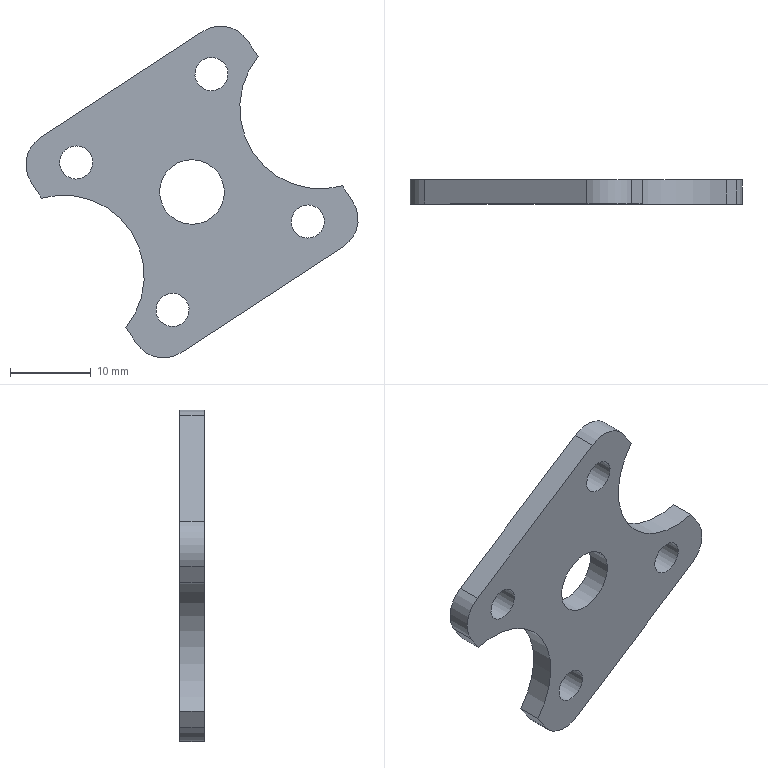Component | SolidWorks | FrontWheelSideThickPlate-2 | 1 solid | 25 faces | box 41.11 x 3 x 41.05 mm | volume 2114 mm3 | cylinder 17 | plane 8 | commonest cylinder face diameters 4.1 x8 8 x6 20 x3
build123d program:
from build123d import *

# Parameters (mm, degrees)
SKETCH1_R           = 2.05
SKETCH1_R_2         = 4
BOSS_EXTRUDE1_DEPTH = 3
FILLET1_R           = 4


with BuildPart() as part:
    # Sketch1 → Boss-Extrude1 (new body)
    with BuildSketch(Plane.XY):
        with BuildLine():
            Line((-16, -9.539), (-16, -15.9))
            Line((-16, -15.9), (16, -15.9))
            Line((16, -15.9), (16, -9.539))
            ThreePointArc((16, -9.539), (9, 0), (16, 9.539))
            Line((16, 9.539), (16, 15.9))
            Line((16, 15.9), (-16, 15.9))
            Line((-16, 15.9), (-16, 9.539))
            ThreePointArc((-16, 9.539), (-10.938, 5.916), (-9, 0))
            ThreePointArc((-9, 0), (-10.938, -5.916), (-16, -9.539))
        make_face()
        with Locations((-10, -10.9)):
            Circle(SKETCH1_R, mode=Mode.SUBTRACT)
        with Locations((10, -10.9)):
            Circle(SKETCH1_R, mode=Mode.SUBTRACT)
        with Locations((-10, 10.9)):
            Circle(SKETCH1_R, mode=Mode.SUBTRACT)
        Circle(SKETCH1_R_2, mode=Mode.SUBTRACT)
        with Locations((10, 10.9)):
            Circle(SKETCH1_R, mode=Mode.SUBTRACT)
    extrude(amount=BOSS_EXTRUDE1_DEPTH)

    # Fillet1
    fillet1_edges = [part.edges().sort_by_distance(p)[0] for p in [
        (-16, 15.9, 1.5),
        (16, 15.9, 1.5),
        (16, -15.9, 1.5),
        (-16, -15.9, 1.5),
    ]]
    fillet(fillet1_edges, radius=FILLET1_R)


solid = part.part

# Placed as in the assembly
solid = solid.moved(Location((0.3183, 23.4, 37), (-90, 0, -33.158)))
STEP:
#1=COLOUR_RGB('',0.7922,0.8196,0.9333);
#2=FILL_AREA_STYLE_COLOUR('',#1);
#3=FILL_AREA_STYLE('',(#2));
#4=SURFACE_STYLE_FILL_AREA(#3);
#5=SURFACE_SIDE_STYLE('',(#4));
#6=SURFACE_STYLE_USAGE(.BOTH.,#5);
#7=PRESENTATION_STYLE_ASSIGNMENT((#6));
#8=CARTESIAN_POINT('',(0.6444,0.9212,1.357));
#9=VERTEX_POINT('',#8);
#10=CARTESIAN_POINT('',(0.5093,0.9212,1.269));
#11=VERTEX_POINT('',#10);
#12=CARTESIAN_POINT('',(0.5768,0.9212,1.313));
#13=DIRECTION('',(0.,1.,0.));
#14=DIRECTION('',(0.8372,0.,0.5469));
#15=AXIS2_PLACEMENT_3D('',#12,#13,#14);
#16=CIRCLE('',#15,0.08071);
#17=EDGE_CURVE('',#9,#11,#16,.T.);
#18=ORIENTED_EDGE('',*,*,#17,.F.);
#19=CARTESIAN_POINT('',(0.6444,1.039,1.357));
#20=VERTEX_POINT('',#19);
#21=CARTESIAN_POINT('',(0.6444,0.9212,1.357));
#22=DIRECTION('',(0.,1.,0.));
#23=VECTOR('',#22,39.37);
#24=LINE('',#21,#23);
#25=EDGE_CURVE('',#9,#20,#24,.T.);
#26=ORIENTED_EDGE('',*,*,#25,.T.);
#27=CARTESIAN_POINT('',(0.5093,1.039,1.269));
#28=VERTEX_POINT('',#27);
#29=CARTESIAN_POINT('',(0.5768,1.039,1.313));
#30=DIRECTION('',(0.,1.,0.));
#31=DIRECTION('',(0.8372,0.,0.5469));
#32=AXIS2_PLACEMENT_3D('',#29,#30,#31);
#33=CIRCLE('',#32,0.08071);
#34=EDGE_CURVE('',#20,#28,#33,.T.);
#35=ORIENTED_EDGE('',*,*,#34,.T.);
#36=CARTESIAN_POINT('',(0.5093,0.9212,1.269));
#37=DIRECTION('',(0.,1.,0.));
#38=VECTOR('',#37,39.37);
#39=LINE('',#36,#38);
#40=EDGE_CURVE('',#11,#28,#39,.T.);
#41=ORIENTED_EDGE('',*,*,#40,.F.);
#42=EDGE_LOOP('',(#18,#26,#35,#41));
#43=FACE_OUTER_BOUND('',#42,.T.);
#44=CARTESIAN_POINT('',(0.5768,0.9212,1.313));
#45=DIRECTION('',(0.,1.,0.));
#46=DIRECTION('',(-0.8372,0.,-0.5469));
#47=AXIS2_PLACEMENT_3D('',#44,#45,#46);
#48=CYLINDRICAL_SURFACE('',#47,0.08071);
#49=ADVANCED_FACE('',(#43),#48,.F.);
#50=CARTESIAN_POINT('',(0.03985,0.9212,1.987));
#51=VERTEX_POINT('',#50);
#52=CARTESIAN_POINT('',(0.175,0.9212,2.075));
#53=VERTEX_POINT('',#52);
#54=CARTESIAN_POINT('',(0.1074,0.9212,2.031));
#55=DIRECTION('',(0.,-1.,0.));
#56=DIRECTION('',(0.8372,0.,0.5469));
#57=AXIS2_PLACEMENT_3D('',#54,#55,#56);
#58=CIRCLE('',#57,0.08071);
#59=EDGE_CURVE('',#51,#53,#58,.T.);
#60=ORIENTED_EDGE('',*,*,#59,.T.);
#61=CARTESIAN_POINT('',(0.175,1.039,2.075));
#62=VERTEX_POINT('',#61);
#63=CARTESIAN_POINT('',(0.175,0.9212,2.075));
#64=DIRECTION('',(0.,1.,0.));
#65=VECTOR('',#64,39.37);
#66=LINE('',#63,#65);
#67=EDGE_CURVE('',#53,#62,#66,.T.);
#68=ORIENTED_EDGE('',*,*,#67,.T.);
#69=CARTESIAN_POINT('',(0.03985,1.039,1.987));
#70=VERTEX_POINT('',#69);
#71=CARTESIAN_POINT('',(0.1074,1.039,2.031));
#72=DIRECTION('',(0.,-1.,0.));
#73=DIRECTION('',(0.8372,0.,0.5469));
#74=AXIS2_PLACEMENT_3D('',#71,#72,#73);
#75=CIRCLE('',#74,0.08071);
#76=EDGE_CURVE('',#70,#62,#75,.T.);
#77=ORIENTED_EDGE('',*,*,#76,.F.);
#78=CARTESIAN_POINT('',(0.03985,0.9212,1.987));
#79=DIRECTION('',(0.,1.,0.));
#80=VECTOR('',#79,39.37);
#81=LINE('',#78,#80);
#82=EDGE_CURVE('',#51,#70,#81,.T.);
#83=ORIENTED_EDGE('',*,*,#82,.F.);
#84=EDGE_LOOP('',(#60,#68,#77,#83));
#85=FACE_OUTER_BOUND('',#84,.T.);
#86=CARTESIAN_POINT('',(0.1074,0.9212,2.031));
#87=DIRECTION('',(0.,1.,0.));
#88=DIRECTION('',(-0.8372,0.,-0.5469));
#89=AXIS2_PLACEMENT_3D('',#86,#87,#88);
#90=CYLINDRICAL_SURFACE('',#89,0.08071);
#91=ADVANCED_FACE('',(#85),#90,.F.);
#92=CARTESIAN_POINT('',(-0.6193,0.9212,1.556));
#93=VERTEX_POINT('',#92);
#94=CARTESIAN_POINT('',(-0.4842,0.9212,1.645));
#95=VERTEX_POINT('',#94);
#96=CARTESIAN_POINT('',(-0.5518,0.9212,1.601));
#97=DIRECTION('',(0.,-1.,0.));
#98=DIRECTION('',(0.8372,0.,0.5469));
#99=AXIS2_PLACEMENT_3D('',#96,#97,#98);
#100=CIRCLE('',#99,0.08071);
#101=EDGE_CURVE('',#93,#95,#100,.T.);
#102=ORIENTED_EDGE('',*,*,#101,.T.);
#103=CARTESIAN_POINT('',(-0.4842,1.039,1.645));
#104=VERTEX_POINT('',#103);
#105=CARTESIAN_POINT('',(-0.4842,0.9212,1.645));
#106=DIRECTION('',(0.,1.,0.));
#107=VECTOR('',#106,39.37);
#108=LINE('',#105,#107);
#109=EDGE_CURVE('',#95,#104,#108,.T.);
#110=ORIENTED_EDGE('',*,*,#109,.T.);
#111=CARTESIAN_POINT('',(-0.6193,1.039,1.556));
#112=VERTEX_POINT('',#111);
#113=CARTESIAN_POINT('',(-0.5518,1.039,1.601));
#114=DIRECTION('',(0.,-1.,0.));
#115=DIRECTION('',(0.8372,0.,0.5469));
#116=AXIS2_PLACEMENT_3D('',#113,#114,#115);
#117=CIRCLE('',#116,0.08071);
#118=EDGE_CURVE('',#112,#104,#117,.T.);
#119=ORIENTED_EDGE('',*,*,#118,.F.);
#120=CARTESIAN_POINT('',(-0.6193,0.9212,1.556));
#121=DIRECTION('',(0.,1.,0.));
#122=VECTOR('',#121,39.37);
#123=LINE('',#120,#122);
#124=EDGE_CURVE('',#93,#112,#123,.T.);
#125=ORIENTED_EDGE('',*,*,#124,.F.);
#126=EDGE_LOOP('',(#102,#110,#119,#125));
#127=FACE_OUTER_BOUND('',#126,.T.);
#128=CARTESIAN_POINT('',(-0.5518,0.9212,1.601));
#129=DIRECTION('',(0.,1.,0.));
#130=DIRECTION('',(-0.8372,0.,-0.5469));
#131=AXIS2_PLACEMENT_3D('',#128,#129,#130);
#132=CYLINDRICAL_SURFACE('',#131,0.08071);
#133=ADVANCED_FACE('',(#127),#132,.F.);
#134=CARTESIAN_POINT('',(-0.01478,0.9212,0.9262));
#135=VERTEX_POINT('',#134);
#136=CARTESIAN_POINT('',(-0.1499,0.9212,0.838));
#137=VERTEX_POINT('',#136);
#138=CARTESIAN_POINT('',(-0.08235,0.9212,0.8821));
#139=DIRECTION('',(0.,1.,0.));
#140=DIRECTION('',(0.8372,0.,0.5469));
#141=AXIS2_PLACEMENT_3D('',#138,#139,#140);
#142=CIRCLE('',#141,0.08071);
#143=EDGE_CURVE('',#135,#137,#142,.T.);
#144=ORIENTED_EDGE('',*,*,#143,.F.);
#145=CARTESIAN_POINT('',(-0.01478,1.039,0.9262));
#146=VERTEX_POINT('',#145);
#147=CARTESIAN_POINT('',(-0.01478,0.9212,0.9262));
#148=DIRECTION('',(0.,1.,0.));
#149=VECTOR('',#148,39.37);
#150=LINE('',#147,#149);
#151=EDGE_CURVE('',#135,#146,#150,.T.);
#152=ORIENTED_EDGE('',*,*,#151,.T.);
#153=CARTESIAN_POINT('',(-0.1499,1.039,0.838));
#154=VERTEX_POINT('',#153);
#155=CARTESIAN_POINT('',(-0.08235,1.039,0.8821));
#156=DIRECTION('',(0.,1.,0.));
#157=DIRECTION('',(0.8372,0.,0.5469));
#158=AXIS2_PLACEMENT_3D('',#155,#156,#157);
#159=CIRCLE('',#158,0.08071);
#160=EDGE_CURVE('',#146,#154,#159,.T.);
#161=ORIENTED_EDGE('',*,*,#160,.T.);
#162=CARTESIAN_POINT('',(-0.1499,0.9212,0.838));
#163=DIRECTION('',(0.,1.,0.));
#164=VECTOR('',#163,39.37);
#165=LINE('',#162,#164);
#166=EDGE_CURVE('',#137,#154,#165,.T.);
#167=ORIENTED_EDGE('',*,*,#166,.F.);
#168=EDGE_LOOP('',(#144,#152,#161,#167));
#169=FACE_OUTER_BOUND('',#168,.T.);
#170=CARTESIAN_POINT('',(-0.08235,0.9212,0.8821));
#171=DIRECTION('',(0.,1.,0.));
#172=DIRECTION('',(-0.8372,0.,-0.5469));
#173=AXIS2_PLACEMENT_3D('',#170,#171,#172);
#174=CYLINDRICAL_SURFACE('',#173,0.08071);
#175=ADVANCED_FACE('',(#169),#174,.F.);
#176=CARTESIAN_POINT('',(-0.1193,0.9212,1.371));
#177=VERTEX_POINT('',#176);
#178=CARTESIAN_POINT('',(0.1444,0.9212,1.543));
#179=VERTEX_POINT('',#178);
#180=CARTESIAN_POINT('',(0.01253,0.9212,1.457));
#181=DIRECTION('',(0.,-1.,0.));
#182=DIRECTION('',(0.8372,0.,0.5469));
#183=AXIS2_PLACEMENT_3D('',#180,#181,#182);
#184=CIRCLE('',#183,0.1575);
#185=EDGE_CURVE('',#177,#179,#184,.T.);
#186=ORIENTED_EDGE('',*,*,#185,.T.);
#187=CARTESIAN_POINT('',(0.1444,1.039,1.543));
#188=VERTEX_POINT('',#187);
#189=CARTESIAN_POINT('',(0.1444,0.9212,1.543));
#190=DIRECTION('',(0.,1.,0.));
#191=VECTOR('',#190,39.37);
#192=LINE('',#189,#191);
#193=EDGE_CURVE('',#179,#188,#192,.T.);
#194=ORIENTED_EDGE('',*,*,#193,.T.);
#195=CARTESIAN_POINT('',(-0.1193,1.039,1.371));
#196=VERTEX_POINT('',#195);
#197=CARTESIAN_POINT('',(0.01253,1.039,1.457));
#198=DIRECTION('',(0.,-1.,0.));
#199=DIRECTION('',(0.8372,0.,0.5469));
#200=AXIS2_PLACEMENT_3D('',#197,#198,#199);
#201=CIRCLE('',#200,0.1575);
#202=EDGE_CURVE('',#196,#188,#201,.T.);
#203=ORIENTED_EDGE('',*,*,#202,.F.);
#204=CARTESIAN_POINT('',(-0.1193,0.9212,1.371));
#205=DIRECTION('',(0.,1.,0.));
#206=VECTOR('',#205,39.37);
#207=LINE('',#204,#206);
#208=EDGE_CURVE('',#177,#196,#207,.T.);
#209=ORIENTED_EDGE('',*,*,#208,.F.);
#210=EDGE_LOOP('',(#186,#194,#203,#209));
#211=FACE_OUTER_BOUND('',#210,.T.);
#212=CARTESIAN_POINT('',(0.01253,0.9212,1.457));
#213=DIRECTION('',(0.,1.,0.));
#214=DIRECTION('',(-0.8372,0.,-0.5469));
#215=AXIS2_PLACEMENT_3D('',#212,#213,#214);
#216=CYLINDRICAL_SURFACE('',#215,0.1575);
#217=ADVANCED_FACE('',(#211),#216,.F.);
#218=CARTESIAN_POINT('',(0.3345,0.9212,2.116));
#219=VERTEX_POINT('',#218);
#220=CARTESIAN_POINT('',(0.3092,0.9212,1.65));
#221=VERTEX_POINT('',#220);
#222=CARTESIAN_POINT('',(0.6388,0.9212,1.866));
#223=DIRECTION('',(0.,-1.,0.));
#224=DIRECTION('',(0.8372,0.,0.5469));
#225=AXIS2_PLACEMENT_3D('',#222,#223,#224);
#226=CIRCLE('',#225,0.3937);
#227=EDGE_CURVE('',#219,#221,#226,.T.);
#228=ORIENTED_EDGE('',*,*,#227,.T.);
#229=CARTESIAN_POINT('',(0.3092,1.039,1.65));
#230=VERTEX_POINT('',#229);
#231=CARTESIAN_POINT('',(0.3092,0.9212,1.65));
#232=DIRECTION('',(0.,1.,0.));
#233=VECTOR('',#232,39.37);
#234=LINE('',#231,#233);
#235=EDGE_CURVE('',#221,#230,#234,.T.);
#236=ORIENTED_EDGE('',*,*,#235,.T.);
#237=CARTESIAN_POINT('',(0.3345,1.039,2.116));
#238=VERTEX_POINT('',#237);
#239=CARTESIAN_POINT('',(0.6388,1.039,1.866));
#240=DIRECTION('',(0.,-1.,0.));
#241=DIRECTION('',(0.8372,0.,0.5469));
#242=AXIS2_PLACEMENT_3D('',#239,#240,#241);
#243=CIRCLE('',#242,0.3937);
#244=EDGE_CURVE('',#238,#230,#243,.T.);
#245=ORIENTED_EDGE('',*,*,#244,.F.);
#246=CARTESIAN_POINT('',(0.3345,0.9212,2.116));
#247=DIRECTION('',(0.,1.,0.));
#248=VECTOR('',#247,39.37);
#249=LINE('',#246,#248);
#250=EDGE_CURVE('',#219,#238,#249,.T.);
#251=ORIENTED_EDGE('',*,*,#250,.F.);
#252=EDGE_LOOP('',(#228,#236,#245,#251));
#253=FACE_OUTER_BOUND('',#252,.T.);
#254=CARTESIAN_POINT('',(0.6388,0.9212,1.866));
#255=DIRECTION('',(0.,1.,0.));
#256=DIRECTION('',(-0.8372,0.,-0.5469));
#257=AXIS2_PLACEMENT_3D('',#254,#255,#256);
#258=CYLINDRICAL_SURFACE('',#257,0.3937);
#259=ADVANCED_FACE('',(#253),#258,.F.);
#260=CARTESIAN_POINT('',(-0.7202,0.9212,1.427));
#261=VERTEX_POINT('',#260);
#262=CARTESIAN_POINT('',(-0.7711,0.9212,1.504));
#263=VERTEX_POINT('',#262);
#264=CARTESIAN_POINT('',(-0.5148,0.9212,1.112));
#265=DIRECTION('',(-0.5469,0.,0.8372));
#266=VECTOR('',#265,39.37);
#267=LINE('',#264,#266);
#268=EDGE_CURVE('',#261,#263,#267,.T.);
#269=ORIENTED_EDGE('',*,*,#268,.T.);
#270=CARTESIAN_POINT('',(-0.7711,1.039,1.504));
#271=VERTEX_POINT('',#270);
#272=CARTESIAN_POINT('',(-0.7711,0.9212,1.504));
#273=DIRECTION('',(0.,1.,0.));
#274=VECTOR('',#273,39.37);
#275=LINE('',#272,#274);
#276=EDGE_CURVE('',#263,#271,#275,.T.);
#277=ORIENTED_EDGE('',*,*,#276,.T.);
#278=CARTESIAN_POINT('',(-0.7202,1.039,1.427));
#279=VERTEX_POINT('',#278);
#280=CARTESIAN_POINT('',(-0.5148,1.039,1.112));
#281=DIRECTION('',(-0.5469,0.,0.8372));
#282=VECTOR('',#281,39.37);
#283=LINE('',#280,#282);
#284=EDGE_CURVE('',#279,#271,#283,.T.);
#285=ORIENTED_EDGE('',*,*,#284,.F.);
#286=CARTESIAN_POINT('',(-0.7202,0.9212,1.427));
#287=DIRECTION('',(0.,1.,0.));
#288=VECTOR('',#287,39.37);
#289=LINE('',#286,#288);
#290=EDGE_CURVE('',#261,#279,#289,.T.);
#291=ORIENTED_EDGE('',*,*,#290,.F.);
#292=EDGE_LOOP('',(#269,#277,#285,#291));
#293=FACE_OUTER_BOUND('',#292,.T.);
#294=CARTESIAN_POINT('',(-0.5148,0.9212,1.112));
#295=DIRECTION('',(-0.8372,0.,-0.5469));
#296=DIRECTION('',(0.,-1.,0.));
#297=AXIS2_PLACEMENT_3D('',#294,#295,#296);
#298=PLANE('',#297);
#299=ADVANCED_FACE('',(#293),#298,.T.);
#300=CARTESIAN_POINT('',(-0.3094,1.039,0.7977));
#301=VERTEX_POINT('',#300);
#302=CARTESIAN_POINT('',(-0.6137,1.039,1.048));
#303=DIRECTION('',(0.,1.,0.));
#304=DIRECTION('',(0.8372,0.,0.5469));
#305=AXIS2_PLACEMENT_3D('',#302,#303,#304);
#306=CIRCLE('',#305,0.3937);
#307=EDGE_CURVE('',#279,#301,#306,.T.);
#308=ORIENTED_EDGE('',*,*,#307,.T.);
#309=CARTESIAN_POINT('',(-0.3094,0.9212,0.7977));
#310=VERTEX_POINT('',#309);
#311=CARTESIAN_POINT('',(-0.3094,0.9212,0.7977));
#312=DIRECTION('',(0.,1.,0.));
#313=VECTOR('',#312,39.37);
#314=LINE('',#311,#313);
#315=EDGE_CURVE('',#310,#301,#314,.T.);
#316=ORIENTED_EDGE('',*,*,#315,.F.);
#317=CARTESIAN_POINT('',(-0.6137,0.9212,1.048));
#318=DIRECTION('',(0.,1.,0.));
#319=DIRECTION('',(0.8372,0.,0.5469));
#320=AXIS2_PLACEMENT_3D('',#317,#318,#319);
#321=CIRCLE('',#320,0.3937);
#322=EDGE_CURVE('',#261,#310,#321,.T.);
#323=ORIENTED_EDGE('',*,*,#322,.F.);
#324=ORIENTED_EDGE('',*,*,#290,.T.);
#325=EDGE_LOOP('',(#308,#316,#323,#324));
#326=FACE_OUTER_BOUND('',#325,.T.);
#327=CARTESIAN_POINT('',(-0.6137,0.9212,1.048));
#328=DIRECTION('',(0.,1.,0.));
#329=DIRECTION('',(-0.8372,0.,-0.5469));
#330=AXIS2_PLACEMENT_3D('',#327,#328,#329);
#331=CYLINDRICAL_SURFACE('',#330,0.3937);
#332=ADVANCED_FACE('',(#326),#331,.F.);
#333=CARTESIAN_POINT('',(-0.2586,1.039,0.7199));
#334=VERTEX_POINT('',#333);
#335=CARTESIAN_POINT('',(-0.5148,1.039,1.112));
#336=DIRECTION('',(-0.5469,0.,0.8372));
#337=VECTOR('',#336,39.37);
#338=LINE('',#335,#337);
#339=EDGE_CURVE('',#334,#301,#338,.T.);
#340=ORIENTED_EDGE('',*,*,#339,.F.);
#341=CARTESIAN_POINT('',(-0.2586,0.9212,0.7199));
#342=VERTEX_POINT('',#341);
#343=CARTESIAN_POINT('',(-0.2586,0.9212,0.7199));
#344=DIRECTION('',(0.,-1.,0.));
#345=VECTOR('',#344,39.37);
#346=LINE('',#343,#345);
#347=EDGE_CURVE('',#334,#342,#346,.T.);
#348=ORIENTED_EDGE('',*,*,#347,.T.);
#349=CARTESIAN_POINT('',(-0.5148,0.9212,1.112));
#350=DIRECTION('',(-0.5469,0.,0.8372));
#351=VECTOR('',#350,39.37);
#352=LINE('',#349,#351);
#353=EDGE_CURVE('',#342,#310,#352,.T.);
#354=ORIENTED_EDGE('',*,*,#353,.T.);
#355=ORIENTED_EDGE('',*,*,#315,.T.);
#356=EDGE_LOOP('',(#340,#348,#354,#355));
#357=FACE_OUTER_BOUND('',#356,.T.);
#358=CARTESIAN_POINT('',(-0.5148,0.9212,1.112));
#359=DIRECTION('',(-0.8372,0.,-0.5469));
#360=DIRECTION('',(0.,-1.,0.));
#361=AXIS2_PLACEMENT_3D('',#358,#359,#360);
#362=PLANE('',#361);
#363=ADVANCED_FACE('',(#357),#362,.T.);
#364=CARTESIAN_POINT('',(-0.0406,0.9212,0.6742));
#365=VERTEX_POINT('',#364);
#366=CARTESIAN_POINT('',(0.7504,0.9212,1.191));
#367=VERTEX_POINT('',#366);
#368=CARTESIAN_POINT('',(0.3549,0.9212,0.9326));
#369=DIRECTION('',(0.8372,0.,0.5469));
#370=VECTOR('',#369,39.37);
#371=LINE('',#368,#370);
#372=EDGE_CURVE('',#365,#367,#371,.T.);
#373=ORIENTED_EDGE('',*,*,#372,.F.);
#374=CARTESIAN_POINT('',(-0.0406,1.039,0.6742));
#375=VERTEX_POINT('',#374);
#376=CARTESIAN_POINT('',(-0.0406,1.039,0.6742));
#377=DIRECTION('',(0.,1.,0.));
#378=VECTOR('',#377,39.37);
#379=LINE('',#376,#378);
#380=EDGE_CURVE('',#365,#375,#379,.T.);
#381=ORIENTED_EDGE('',*,*,#380,.T.);
#382=CARTESIAN_POINT('',(0.7504,1.039,1.191));
#383=VERTEX_POINT('',#382);
#384=CARTESIAN_POINT('',(0.3549,1.039,0.9326));
#385=DIRECTION('',(0.8372,0.,0.5469));
#386=VECTOR('',#385,39.37);
#387=LINE('',#384,#386);
#388=EDGE_CURVE('',#375,#383,#387,.T.);
#389=ORIENTED_EDGE('',*,*,#388,.T.);
#390=CARTESIAN_POINT('',(0.7504,0.9212,1.191));
#391=DIRECTION('',(0.,-1.,0.));
#392=VECTOR('',#391,39.37);
#393=LINE('',#390,#392);
#394=EDGE_CURVE('',#383,#367,#393,.T.);
#395=ORIENTED_EDGE('',*,*,#394,.T.);
#396=EDGE_LOOP('',(#373,#381,#389,#395));
#397=FACE_OUTER_BOUND('',#396,.T.);
#398=CARTESIAN_POINT('',(0.3549,0.9212,0.9326));
#399=DIRECTION('',(-0.5469,0.,0.8372));
#400=DIRECTION('',(-0.8372,0.,-0.5469));
#401=AXIS2_PLACEMENT_3D('',#398,#399,#400);
#402=PLANE('',#401);
#403=ADVANCED_FACE('',(#397),#402,.F.);
#404=CARTESIAN_POINT('',(0.7961,0.9212,1.409));
#405=VERTEX_POINT('',#404);
#406=CARTESIAN_POINT('',(0.7453,0.9212,1.487));
#407=VERTEX_POINT('',#406);
#408=CARTESIAN_POINT('',(0.5399,0.9212,1.801));
#409=DIRECTION('',(-0.5469,0.,0.8372));
#410=VECTOR('',#409,39.37);
#411=LINE('',#408,#410);
#412=EDGE_CURVE('',#405,#407,#411,.T.);
#413=ORIENTED_EDGE('',*,*,#412,.F.);
#414=CARTESIAN_POINT('',(0.7961,1.039,1.409));
#415=VERTEX_POINT('',#414);
#416=CARTESIAN_POINT('',(0.7961,0.9212,1.409));
#417=DIRECTION('',(0.,1.,0.));
#418=VECTOR('',#417,39.37);
#419=LINE('',#416,#418);
#420=EDGE_CURVE('',#405,#415,#419,.T.);
#421=ORIENTED_EDGE('',*,*,#420,.T.);
#422=CARTESIAN_POINT('',(0.7453,1.039,1.487));
#423=VERTEX_POINT('',#422);
#424=CARTESIAN_POINT('',(0.5399,1.039,1.801));
#425=DIRECTION('',(-0.5469,0.,0.8372));
#426=VECTOR('',#425,39.37);
#427=LINE('',#424,#426);
#428=EDGE_CURVE('',#415,#423,#427,.T.);
#429=ORIENTED_EDGE('',*,*,#428,.T.);
#430=CARTESIAN_POINT('',(0.7453,0.9212,1.487));
#431=DIRECTION('',(0.,1.,0.));
#432=VECTOR('',#431,39.37);
#433=LINE('',#430,#432);
#434=EDGE_CURVE('',#407,#423,#433,.T.);
#435=ORIENTED_EDGE('',*,*,#434,.F.);
#436=EDGE_LOOP('',(#413,#421,#429,#435));
#437=FACE_OUTER_BOUND('',#436,.T.);
#438=CARTESIAN_POINT('',(0.5399,0.9212,1.801));
#439=DIRECTION('',(-0.8372,0.,-0.5469));
#440=DIRECTION('',(0.5469,0.,-0.8372));
#441=AXIS2_PLACEMENT_3D('',#438,#439,#440);
#442=PLANE('',#441);
#443=ADVANCED_FACE('',(#437),#442,.F.);
#444=ORIENTED_EDGE('',*,*,#235,.F.);
#445=CARTESIAN_POINT('',(0.6388,0.9212,1.866));
#446=DIRECTION('',(0.,-1.,0.));
#447=DIRECTION('',(0.8372,0.,0.5469));
#448=AXIS2_PLACEMENT_3D('',#445,#446,#447);
#449=CIRCLE('',#448,0.3937);
#450=EDGE_CURVE('',#221,#407,#449,.T.);
#451=ORIENTED_EDGE('',*,*,#450,.T.);
#452=ORIENTED_EDGE('',*,*,#434,.T.);
#453=CARTESIAN_POINT('',(0.6388,1.039,1.866));
#454=DIRECTION('',(0.,-1.,0.));
#455=DIRECTION('',(0.8372,0.,0.5469));
#456=AXIS2_PLACEMENT_3D('',#453,#454,#455);
#457=CIRCLE('',#456,0.3937);
#458=EDGE_CURVE('',#230,#423,#457,.T.);
#459=ORIENTED_EDGE('',*,*,#458,.F.);
#460=EDGE_LOOP('',(#444,#451,#452,#459));
#461=FACE_OUTER_BOUND('',#460,.T.);
#462=CARTESIAN_POINT('',(0.6388,0.9212,1.866));
#463=DIRECTION('',(0.,1.,0.));
#464=DIRECTION('',(-0.8372,0.,-0.5469));
#465=AXIS2_PLACEMENT_3D('',#462,#463,#464);
#466=CYLINDRICAL_SURFACE('',#465,0.3937);
#467=ADVANCED_FACE('',(#461),#466,.F.);
#468=CARTESIAN_POINT('',(0.2836,1.039,2.193));
#469=VERTEX_POINT('',#468);
#470=CARTESIAN_POINT('',(0.5399,1.039,1.801));
#471=DIRECTION('',(-0.5469,0.,0.8372));
#472=VECTOR('',#471,39.37);
#473=LINE('',#470,#472);
#474=EDGE_CURVE('',#238,#469,#473,.T.);
#475=ORIENTED_EDGE('',*,*,#474,.T.);
#476=CARTESIAN_POINT('',(0.2836,0.9212,2.193));
#477=VERTEX_POINT('',#476);
#478=CARTESIAN_POINT('',(0.2836,0.9212,2.193));
#479=DIRECTION('',(0.,-1.,0.));
#480=VECTOR('',#479,39.37);
#481=LINE('',#478,#480);
#482=EDGE_CURVE('',#469,#477,#481,.T.);
#483=ORIENTED_EDGE('',*,*,#482,.T.);
#484=CARTESIAN_POINT('',(0.5399,0.9212,1.801));
#485=DIRECTION('',(-0.5469,0.,0.8372));
#486=VECTOR('',#485,39.37);
#487=LINE('',#484,#486);
#488=EDGE_CURVE('',#219,#477,#487,.T.);
#489=ORIENTED_EDGE('',*,*,#488,.F.);
#490=ORIENTED_EDGE('',*,*,#250,.T.);
#491=EDGE_LOOP('',(#475,#483,#489,#490));
#492=FACE_OUTER_BOUND('',#491,.T.);
#493=CARTESIAN_POINT('',(0.5399,0.9212,1.801));
#494=DIRECTION('',(-0.8372,0.,-0.5469));
#495=DIRECTION('',(0.5469,0.,-0.8372));
#496=AXIS2_PLACEMENT_3D('',#493,#494,#495);
#497=PLANE('',#496);
#498=ADVANCED_FACE('',(#492),#497,.F.);
#499=ORIENTED_EDGE('',*,*,#193,.F.);
#500=CARTESIAN_POINT('',(0.01253,0.9212,1.457));
#501=DIRECTION('',(0.,-1.,0.));
#502=DIRECTION('',(0.8372,0.,0.5469));
#503=AXIS2_PLACEMENT_3D('',#500,#501,#502);
#504=CIRCLE('',#503,0.1575);
#505=EDGE_CURVE('',#179,#177,#504,.T.);
#506=ORIENTED_EDGE('',*,*,#505,.T.);
#507=ORIENTED_EDGE('',*,*,#208,.T.);
#508=CARTESIAN_POINT('',(0.01253,1.039,1.457));
#509=DIRECTION('',(0.,-1.,0.));
#510=DIRECTION('',(0.8372,0.,0.5469));
#511=AXIS2_PLACEMENT_3D('',#508,#509,#510);
#512=CIRCLE('',#511,0.1575);
#513=EDGE_CURVE('',#188,#196,#512,.T.);
#514=ORIENTED_EDGE('',*,*,#513,.F.);
#515=EDGE_LOOP('',(#499,#506,#507,#514));
#516=FACE_OUTER_BOUND('',#515,.T.);
#517=CARTESIAN_POINT('',(0.01253,0.9212,1.457));
#518=DIRECTION('',(0.,1.,0.));
#519=DIRECTION('',(-0.8372,0.,-0.5469));
#520=AXIS2_PLACEMENT_3D('',#517,#518,#519);
#521=CYLINDRICAL_SURFACE('',#520,0.1575);
#522=ADVANCED_FACE('',(#516),#521,.F.);
#523=ORIENTED_EDGE('',*,*,#151,.F.);
#524=CARTESIAN_POINT('',(-0.08235,0.9212,0.8821));
#525=DIRECTION('',(0.,1.,0.));
#526=DIRECTION('',(0.8372,0.,0.5469));
#527=AXIS2_PLACEMENT_3D('',#524,#525,#526);
#528=CIRCLE('',#527,0.08071);
#529=EDGE_CURVE('',#137,#135,#528,.T.);
#530=ORIENTED_EDGE('',*,*,#529,.F.);
#531=ORIENTED_EDGE('',*,*,#166,.T.);
#532=CARTESIAN_POINT('',(-0.08235,1.039,0.8821));
#533=DIRECTION('',(0.,1.,0.));
#534=DIRECTION('',(0.8372,0.,0.5469));
#535=AXIS2_PLACEMENT_3D('',#532,#533,#534);
#536=CIRCLE('',#535,0.08071);
#537=EDGE_CURVE('',#154,#146,#536,.T.);
#538=ORIENTED_EDGE('',*,*,#537,.T.);
#539=EDGE_LOOP('',(#523,#530,#531,#538));
#540=FACE_OUTER_BOUND('',#539,.T.);
#541=CARTESIAN_POINT('',(-0.08235,0.9212,0.8821));
#542=DIRECTION('',(0.,1.,0.));
#543=DIRECTION('',(-0.8372,0.,-0.5469));
#544=AXIS2_PLACEMENT_3D('',#541,#542,#543);
#545=CYLINDRICAL_SURFACE('',#544,0.08071);
#546=ADVANCED_FACE('',(#540),#545,.F.);
#547=ORIENTED_EDGE('',*,*,#109,.F.);
#548=CARTESIAN_POINT('',(-0.5518,0.9212,1.601));
#549=DIRECTION('',(0.,-1.,0.));
#550=DIRECTION('',(0.8372,0.,0.5469));
#551=AXIS2_PLACEMENT_3D('',#548,#549,#550);
#552=CIRCLE('',#551,0.08071);
#553=EDGE_CURVE('',#95,#93,#552,.T.);
#554=ORIENTED_EDGE('',*,*,#553,.T.);
#555=ORIENTED_EDGE('',*,*,#124,.T.);
#556=CARTESIAN_POINT('',(-0.5518,1.039,1.601));
#557=DIRECTION('',(0.,-1.,0.));
#558=DIRECTION('',(0.8372,0.,0.5469));
#559=AXIS2_PLACEMENT_3D('',#556,#557,#558);
#560=CIRCLE('',#559,0.08071);
#561=EDGE_CURVE('',#104,#112,#560,.T.);
#562=ORIENTED_EDGE('',*,*,#561,.F.);
#563=EDGE_LOOP('',(#547,#554,#555,#562));
#564=FACE_OUTER_BOUND('',#563,.T.);
#565=CARTESIAN_POINT('',(-0.5518,0.9212,1.601));
#566=DIRECTION('',(0.,1.,0.));
#567=DIRECTION('',(-0.8372,0.,-0.5469));
#568=AXIS2_PLACEMENT_3D('',#565,#566,#567);
#569=CYLINDRICAL_SURFACE('',#568,0.08071);
#570=ADVANCED_FACE('',(#564),#569,.F.);
#571=ORIENTED_EDGE('',*,*,#67,.F.);
#572=CARTESIAN_POINT('',(0.1074,0.9212,2.031));
#573=DIRECTION('',(0.,-1.,0.));
#574=DIRECTION('',(0.8372,0.,0.5469));
#575=AXIS2_PLACEMENT_3D('',#572,#573,#574);
#576=CIRCLE('',#575,0.08071);
#577=EDGE_CURVE('',#53,#51,#576,.T.);
#578=ORIENTED_EDGE('',*,*,#577,.T.);
#579=ORIENTED_EDGE('',*,*,#82,.T.);
#580=CARTESIAN_POINT('',(0.1074,1.039,2.031));
#581=DIRECTION('',(0.,-1.,0.));
#582=DIRECTION('',(0.8372,0.,0.5469));
#583=AXIS2_PLACEMENT_3D('',#580,#581,#582);
#584=CIRCLE('',#583,0.08071);
#585=EDGE_CURVE('',#62,#70,#584,.T.);
#586=ORIENTED_EDGE('',*,*,#585,.F.);
#587=EDGE_LOOP('',(#571,#578,#579,#586));
#588=FACE_OUTER_BOUND('',#587,.T.);
#589=CARTESIAN_POINT('',(0.1074,0.9212,2.031));
#590=DIRECTION('',(0.,1.,0.));
#591=DIRECTION('',(-0.8372,0.,-0.5469));
#592=AXIS2_PLACEMENT_3D('',#589,#590,#591);
#593=CYLINDRICAL_SURFACE('',#592,0.08071);
#594=ADVANCED_FACE('',(#588),#593,.F.);
#595=ORIENTED_EDGE('',*,*,#25,.F.);
#596=CARTESIAN_POINT('',(0.5768,0.9212,1.313));
#597=DIRECTION('',(0.,1.,0.));
#598=DIRECTION('',(0.8372,0.,0.5469));
#599=AXIS2_PLACEMENT_3D('',#596,#597,#598);
#600=CIRCLE('',#599,0.08071);
#601=EDGE_CURVE('',#11,#9,#600,.T.);
#602=ORIENTED_EDGE('',*,*,#601,.F.);
#603=ORIENTED_EDGE('',*,*,#40,.T.);
#604=CARTESIAN_POINT('',(0.5768,1.039,1.313));
#605=DIRECTION('',(0.,1.,0.));
#606=DIRECTION('',(0.8372,0.,0.5469));
#607=AXIS2_PLACEMENT_3D('',#604,#605,#606);
#608=CIRCLE('',#607,0.08071);
#609=EDGE_CURVE('',#28,#20,#608,.T.);
#610=ORIENTED_EDGE('',*,*,#609,.T.);
#611=EDGE_LOOP('',(#595,#602,#603,#610));
#612=FACE_OUTER_BOUND('',#611,.T.);
#613=CARTESIAN_POINT('',(0.5768,0.9212,1.313));
#614=DIRECTION('',(0.,1.,0.));
#615=DIRECTION('',(-0.8372,0.,-0.5469));
#616=AXIS2_PLACEMENT_3D('',#613,#614,#615);
#617=CYLINDRICAL_SURFACE('',#616,0.08071);
#618=ADVANCED_FACE('',(#612),#617,.F.);
#619=CARTESIAN_POINT('',(-0.7254,0.9212,1.722));
#620=VERTEX_POINT('',#619);
#621=CARTESIAN_POINT('',(0.06567,0.9212,2.239));
#622=VERTEX_POINT('',#621);
#623=CARTESIAN_POINT('',(-0.3298,0.9212,1.981));
#624=DIRECTION('',(0.8372,0.,0.5469));
#625=VECTOR('',#624,39.37);
#626=LINE('',#623,#625);
#627=EDGE_CURVE('',#620,#622,#626,.T.);
#628=ORIENTED_EDGE('',*,*,#627,.T.);
#629=CARTESIAN_POINT('',(0.06567,1.039,2.239));
#630=VERTEX_POINT('',#629);
#631=CARTESIAN_POINT('',(0.06567,1.039,2.239));
#632=DIRECTION('',(0.,1.,0.));
#633=VECTOR('',#632,39.37);
#634=LINE('',#631,#633);
#635=EDGE_CURVE('',#622,#630,#634,.T.);
#636=ORIENTED_EDGE('',*,*,#635,.T.);
#637=CARTESIAN_POINT('',(-0.7254,1.039,1.722));
#638=VERTEX_POINT('',#637);
#639=CARTESIAN_POINT('',(-0.3298,1.039,1.981));
#640=DIRECTION('',(0.8372,0.,0.5469));
#641=VECTOR('',#640,39.37);
#642=LINE('',#639,#641);
#643=EDGE_CURVE('',#638,#630,#642,.T.);
#644=ORIENTED_EDGE('',*,*,#643,.F.);
#645=CARTESIAN_POINT('',(-0.7254,0.9212,1.722));
#646=DIRECTION('',(0.,-1.,0.));
#647=VECTOR('',#646,39.37);
#648=LINE('',#645,#647);
#649=EDGE_CURVE('',#638,#620,#648,.T.);
#650=ORIENTED_EDGE('',*,*,#649,.T.);
#651=EDGE_LOOP('',(#628,#636,#644,#650));
#652=FACE_OUTER_BOUND('',#651,.T.);
#653=CARTESIAN_POINT('',(-0.3298,0.9212,1.981));
#654=DIRECTION('',(-0.5469,0.,0.8372));
#655=DIRECTION('',(-0.8372,0.,-0.5469));
#656=AXIS2_PLACEMENT_3D('',#653,#654,#655);
#657=PLANE('',#656);
#658=ADVANCED_FACE('',(#652),#657,.T.);
#659=ORIENTED_EDGE('',*,*,#601,.T.);
#660=ORIENTED_EDGE('',*,*,#17,.T.);
#661=EDGE_LOOP('',(#659,#660));
#662=FACE_BOUND('',#661,.T.);
#663=ORIENTED_EDGE('',*,*,#59,.F.);
#664=ORIENTED_EDGE('',*,*,#577,.F.);
#665=EDGE_LOOP('',(#663,#664));
#666=FACE_BOUND('',#665,.T.);
#667=ORIENTED_EDGE('',*,*,#101,.F.);
#668=ORIENTED_EDGE('',*,*,#553,.F.);
#669=EDGE_LOOP('',(#667,#668));
#670=FACE_BOUND('',#669,.T.);
#671=ORIENTED_EDGE('',*,*,#529,.T.);
#672=ORIENTED_EDGE('',*,*,#143,.T.);
#673=EDGE_LOOP('',(#671,#672));
#674=FACE_BOUND('',#673,.T.);
#675=ORIENTED_EDGE('',*,*,#185,.F.);
#676=ORIENTED_EDGE('',*,*,#505,.F.);
#677=EDGE_LOOP('',(#675,#676));
#678=FACE_BOUND('',#677,.T.);
#679=ORIENTED_EDGE('',*,*,#353,.F.);
#680=CARTESIAN_POINT('',(-0.1267,0.9212,0.8061));
#681=DIRECTION('',(0.,-1.,0.));
#682=DIRECTION('',(0.8372,0.,0.5469));
#683=AXIS2_PLACEMENT_3D('',#680,#681,#682);
#684=CIRCLE('',#683,0.1575);
#685=EDGE_CURVE('',#342,#365,#684,.T.);
#686=ORIENTED_EDGE('',*,*,#685,.T.);
#687=ORIENTED_EDGE('',*,*,#372,.T.);
#688=CARTESIAN_POINT('',(0.6643,0.9212,1.323));
#689=DIRECTION('',(0.,-1.,0.));
#690=DIRECTION('',(0.8372,0.,0.5469));
#691=AXIS2_PLACEMENT_3D('',#688,#689,#690);
#692=CIRCLE('',#691,0.1575);
#693=EDGE_CURVE('',#367,#405,#692,.T.);
#694=ORIENTED_EDGE('',*,*,#693,.T.);
#695=ORIENTED_EDGE('',*,*,#412,.T.);
#696=ORIENTED_EDGE('',*,*,#450,.F.);
#697=ORIENTED_EDGE('',*,*,#227,.F.);
#698=ORIENTED_EDGE('',*,*,#488,.T.);
#699=CARTESIAN_POINT('',(0.1518,0.9212,2.107));
#700=DIRECTION('',(0.,-1.,0.));
#701=DIRECTION('',(0.8372,0.,0.5469));
#702=AXIS2_PLACEMENT_3D('',#699,#700,#701);
#703=CIRCLE('',#702,0.1575);
#704=EDGE_CURVE('',#477,#622,#703,.T.);
#705=ORIENTED_EDGE('',*,*,#704,.T.);
#706=ORIENTED_EDGE('',*,*,#627,.F.);
#707=CARTESIAN_POINT('',(-0.6392,0.9212,1.591));
#708=DIRECTION('',(0.,-1.,0.));
#709=DIRECTION('',(0.8372,0.,0.5469));
#710=AXIS2_PLACEMENT_3D('',#707,#708,#709);
#711=CIRCLE('',#710,0.1575);
#712=EDGE_CURVE('',#620,#263,#711,.T.);
#713=ORIENTED_EDGE('',*,*,#712,.T.);
#714=ORIENTED_EDGE('',*,*,#268,.F.);
#715=ORIENTED_EDGE('',*,*,#322,.T.);
#716=EDGE_LOOP('',(#679,#686,#687,#694,#695,#696,#697,#698,#705,#706,#713,#714,#715));
#717=FACE_OUTER_BOUND('',#716,.T.);
#718=CARTESIAN_POINT('',(0.01253,0.9212,1.457));
#719=DIRECTION('',(0.,-1.,0.));
#720=DIRECTION('',(0.8372,0.,0.5469));
#721=AXIS2_PLACEMENT_3D('',#718,#719,#720);
#722=PLANE('',#721);
#723=ADVANCED_FACE('',(#662,#666,#670,#674,#678,#717),#722,.T.);
#724=ORIENTED_EDGE('',*,*,#609,.F.);
#725=ORIENTED_EDGE('',*,*,#34,.F.);
#726=EDGE_LOOP('',(#724,#725));
#727=FACE_BOUND('',#726,.T.);
#728=ORIENTED_EDGE('',*,*,#76,.T.);
#729=ORIENTED_EDGE('',*,*,#585,.T.);
#730=EDGE_LOOP('',(#728,#729));
#731=FACE_BOUND('',#730,.T.);
#732=ORIENTED_EDGE('',*,*,#118,.T.);
#733=ORIENTED_EDGE('',*,*,#561,.T.);
#734=EDGE_LOOP('',(#732,#733));
#735=FACE_BOUND('',#734,.T.);
#736=ORIENTED_EDGE('',*,*,#537,.F.);
#737=ORIENTED_EDGE('',*,*,#160,.F.);
#738=EDGE_LOOP('',(#736,#737));
#739=FACE_BOUND('',#738,.T.);
#740=ORIENTED_EDGE('',*,*,#202,.T.);
#741=ORIENTED_EDGE('',*,*,#513,.T.);
#742=EDGE_LOOP('',(#740,#741));
#743=FACE_BOUND('',#742,.T.);
#744=ORIENTED_EDGE('',*,*,#388,.F.);
#745=CARTESIAN_POINT('',(-0.1267,1.039,0.8061));
#746=DIRECTION('',(0.,1.,0.));
#747=DIRECTION('',(0.8372,0.,0.5469));
#748=AXIS2_PLACEMENT_3D('',#745,#746,#747);
#749=CIRCLE('',#748,0.1575);
#750=EDGE_CURVE('',#375,#334,#749,.T.);
#751=ORIENTED_EDGE('',*,*,#750,.T.);
#752=ORIENTED_EDGE('',*,*,#339,.T.);
#753=ORIENTED_EDGE('',*,*,#307,.F.);
#754=ORIENTED_EDGE('',*,*,#284,.T.);
#755=CARTESIAN_POINT('',(-0.6392,1.039,1.591));
#756=DIRECTION('',(0.,1.,0.));
#757=DIRECTION('',(0.8372,0.,0.5469));
#758=AXIS2_PLACEMENT_3D('',#755,#756,#757);
#759=CIRCLE('',#758,0.1575);
#760=EDGE_CURVE('',#271,#638,#759,.T.);
#761=ORIENTED_EDGE('',*,*,#760,.T.);
#762=ORIENTED_EDGE('',*,*,#643,.T.);
#763=CARTESIAN_POINT('',(0.1518,1.039,2.107));
#764=DIRECTION('',(0.,1.,0.));
#765=DIRECTION('',(0.8372,0.,0.5469));
#766=AXIS2_PLACEMENT_3D('',#763,#764,#765);
#767=CIRCLE('',#766,0.1575);
#768=EDGE_CURVE('',#630,#469,#767,.T.);
#769=ORIENTED_EDGE('',*,*,#768,.T.);
#770=ORIENTED_EDGE('',*,*,#474,.F.);
#771=ORIENTED_EDGE('',*,*,#244,.T.);
#772=ORIENTED_EDGE('',*,*,#458,.T.);
#773=ORIENTED_EDGE('',*,*,#428,.F.);
#774=CARTESIAN_POINT('',(0.6643,1.039,1.323));
#775=DIRECTION('',(0.,1.,0.));
#776=DIRECTION('',(0.8372,0.,0.5469));
#777=AXIS2_PLACEMENT_3D('',#774,#775,#776);
#778=CIRCLE('',#777,0.1575);
#779=EDGE_CURVE('',#415,#383,#778,.T.);
#780=ORIENTED_EDGE('',*,*,#779,.T.);
#781=EDGE_LOOP('',(#744,#751,#752,#753,#754,#761,#762,#769,#770,#771,#772,#773,#780));
#782=FACE_OUTER_BOUND('',#781,.T.);
#783=CARTESIAN_POINT('',(0.01253,1.039,1.457));
#784=DIRECTION('',(0.,-1.,0.));
#785=DIRECTION('',(0.8372,0.,0.5469));
#786=AXIS2_PLACEMENT_3D('',#783,#784,#785);
#787=PLANE('',#786);
#788=ADVANCED_FACE('',(#727,#731,#735,#739,#743,#782),#787,.F.);
#789=ORIENTED_EDGE('',*,*,#685,.F.);
#790=ORIENTED_EDGE('',*,*,#347,.F.);
#791=ORIENTED_EDGE('',*,*,#750,.F.);
#792=ORIENTED_EDGE('',*,*,#380,.F.);
#793=EDGE_LOOP('',(#789,#790,#791,#792));
#794=FACE_OUTER_BOUND('',#793,.T.);
#795=CARTESIAN_POINT('',(-0.1267,0.9212,0.8061));
#796=DIRECTION('',(0.,-1.,0.));
#797=DIRECTION('',(0.8372,0.,0.5469));
#798=AXIS2_PLACEMENT_3D('',#795,#796,#797);
#799=CYLINDRICAL_SURFACE('',#798,0.1575);
#800=ADVANCED_FACE('',(#794),#799,.T.);
#801=ORIENTED_EDGE('',*,*,#693,.F.);
#802=ORIENTED_EDGE('',*,*,#394,.F.);
#803=ORIENTED_EDGE('',*,*,#779,.F.);
#804=ORIENTED_EDGE('',*,*,#420,.F.);
#805=EDGE_LOOP('',(#801,#802,#803,#804));
#806=FACE_OUTER_BOUND('',#805,.T.);
#807=CARTESIAN_POINT('',(0.6643,0.9212,1.323));
#808=DIRECTION('',(0.,1.,0.));
#809=DIRECTION('',(-0.8372,0.,-0.5469));
#810=AXIS2_PLACEMENT_3D('',#807,#808,#809);
#811=CYLINDRICAL_SURFACE('',#810,0.1575);
#812=ADVANCED_FACE('',(#806),#811,.T.);
#813=ORIENTED_EDGE('',*,*,#704,.F.);
#814=ORIENTED_EDGE('',*,*,#482,.F.);
#815=ORIENTED_EDGE('',*,*,#768,.F.);
#816=ORIENTED_EDGE('',*,*,#635,.F.);
#817=EDGE_LOOP('',(#813,#814,#815,#816));
#818=FACE_OUTER_BOUND('',#817,.T.);
#819=CARTESIAN_POINT('',(0.1518,0.9212,2.107));
#820=DIRECTION('',(0.,-1.,0.));
#821=DIRECTION('',(0.8372,0.,0.5469));
#822=AXIS2_PLACEMENT_3D('',#819,#820,#821);
#823=CYLINDRICAL_SURFACE('',#822,0.1575);
#824=ADVANCED_FACE('',(#818),#823,.T.);
#825=ORIENTED_EDGE('',*,*,#712,.F.);
#826=ORIENTED_EDGE('',*,*,#649,.F.);
#827=ORIENTED_EDGE('',*,*,#760,.F.);
#828=ORIENTED_EDGE('',*,*,#276,.F.);
#829=EDGE_LOOP('',(#825,#826,#827,#828));
#830=FACE_OUTER_BOUND('',#829,.T.);
#831=CARTESIAN_POINT('',(-0.6392,0.9212,1.591));
#832=DIRECTION('',(0.,1.,0.));
#833=DIRECTION('',(-0.8372,0.,-0.5469));
#834=AXIS2_PLACEMENT_3D('',#831,#832,#833);
#835=CYLINDRICAL_SURFACE('',#834,0.1575);
#836=ADVANCED_FACE('',(#830),#835,.T.);
#837=CLOSED_SHELL('',(#49,#91,#133,#175,#217,#259,#299,#332,#363,#403,#443,#467,#498,#522,#546,#570,#594,#618,#658,#723,#788,#800,#812,#824,#836));
#838=MANIFOLD_SOLID_BREP('',#837);
#839=STYLED_ITEM('',(#7),#838);
#840=(LENGTH_UNIT()NAMED_UNIT(*)SI_UNIT($,.METRE.));
#841=LENGTH_MEASURE_WITH_UNIT(LENGTH_MEASURE(0.0254),#840);
#842=DIMENSIONAL_EXPONENTS(1.,0.,0.,0.,0.,0.,0.);
#843=(CONVERSION_BASED_UNIT('',#841)LENGTH_UNIT()NAMED_UNIT(#842));
#844=UNCERTAINTY_MEASURE_WITH_UNIT(LENGTH_MEASURE(0.00001),#843,'','');
#845=(NAMED_UNIT(*)PLANE_ANGLE_UNIT()SI_UNIT($,.RADIAN.));
#846=(NAMED_UNIT(*)SI_UNIT($,.STERADIAN.)SOLID_ANGLE_UNIT());
#847=(GEOMETRIC_REPRESENTATION_CONTEXT(3)GLOBAL_UNCERTAINTY_ASSIGNED_CONTEXT((#844))GLOBAL_UNIT_ASSIGNED_CONTEXT((#843,#845,#846))REPRESENTATION_CONTEXT('',''));
#848=MECHANICAL_DESIGN_GEOMETRIC_PRESENTATION_REPRESENTATION('',(#839),#847);
#849=PRESENTATION_LAYER_ASSIGNMENT('','',(#839));
#850=CARTESIAN_POINT('',(0.,0.,0.));
#851=DIRECTION('',(0.,0.,1.));
#852=DIRECTION('',(1.,0.,0.));
#853=AXIS2_PLACEMENT_3D('',#850,#851,#852);
#854=(LENGTH_UNIT()NAMED_UNIT(*)SI_UNIT($,.METRE.));
#855=LENGTH_MEASURE_WITH_UNIT(LENGTH_MEASURE(0.0254),#854);
#856=DIMENSIONAL_EXPONENTS(1.,0.,0.,0.,0.,0.,0.);
#857=(CONVERSION_BASED_UNIT('',#855)LENGTH_UNIT()NAMED_UNIT(#856));
#858=UNCERTAINTY_MEASURE_WITH_UNIT(LENGTH_MEASURE(0.00001),#857,'','');
#859=(NAMED_UNIT(*)PLANE_ANGLE_UNIT()SI_UNIT($,.RADIAN.));
#860=(NAMED_UNIT(*)SI_UNIT($,.STERADIAN.)SOLID_ANGLE_UNIT());
#861=(GEOMETRIC_REPRESENTATION_CONTEXT(3)GLOBAL_UNCERTAINTY_ASSIGNED_CONTEXT((#858))GLOBAL_UNIT_ASSIGNED_CONTEXT((#857,#859,#860))REPRESENTATION_CONTEXT('',''));
#862=ADVANCED_BREP_SHAPE_REPRESENTATION('',(#838,#853),#861);